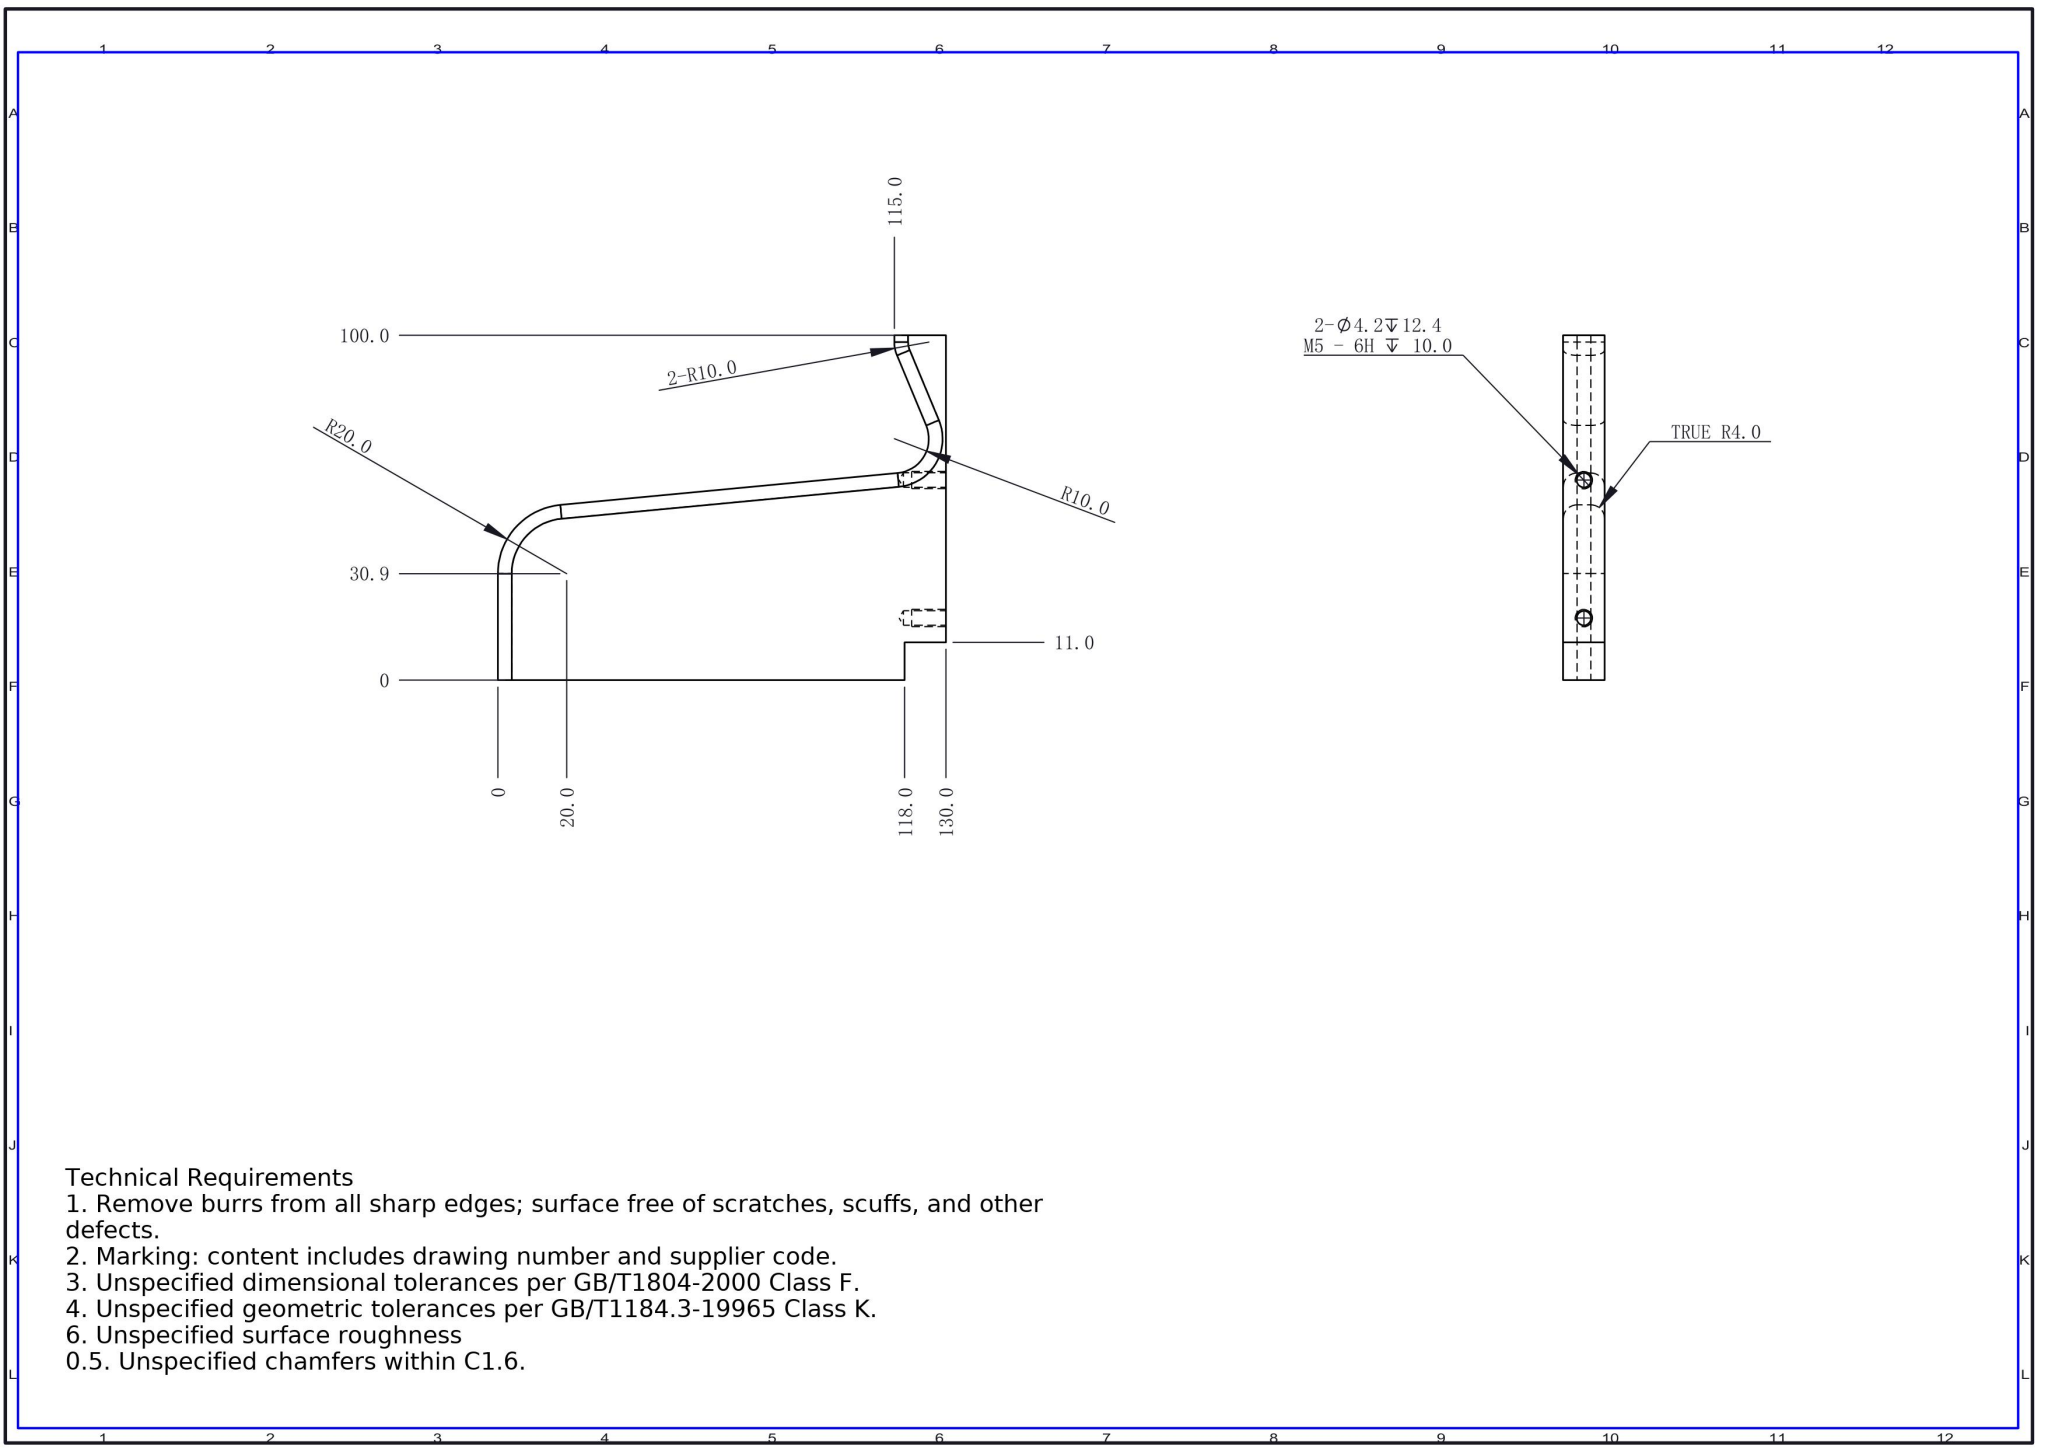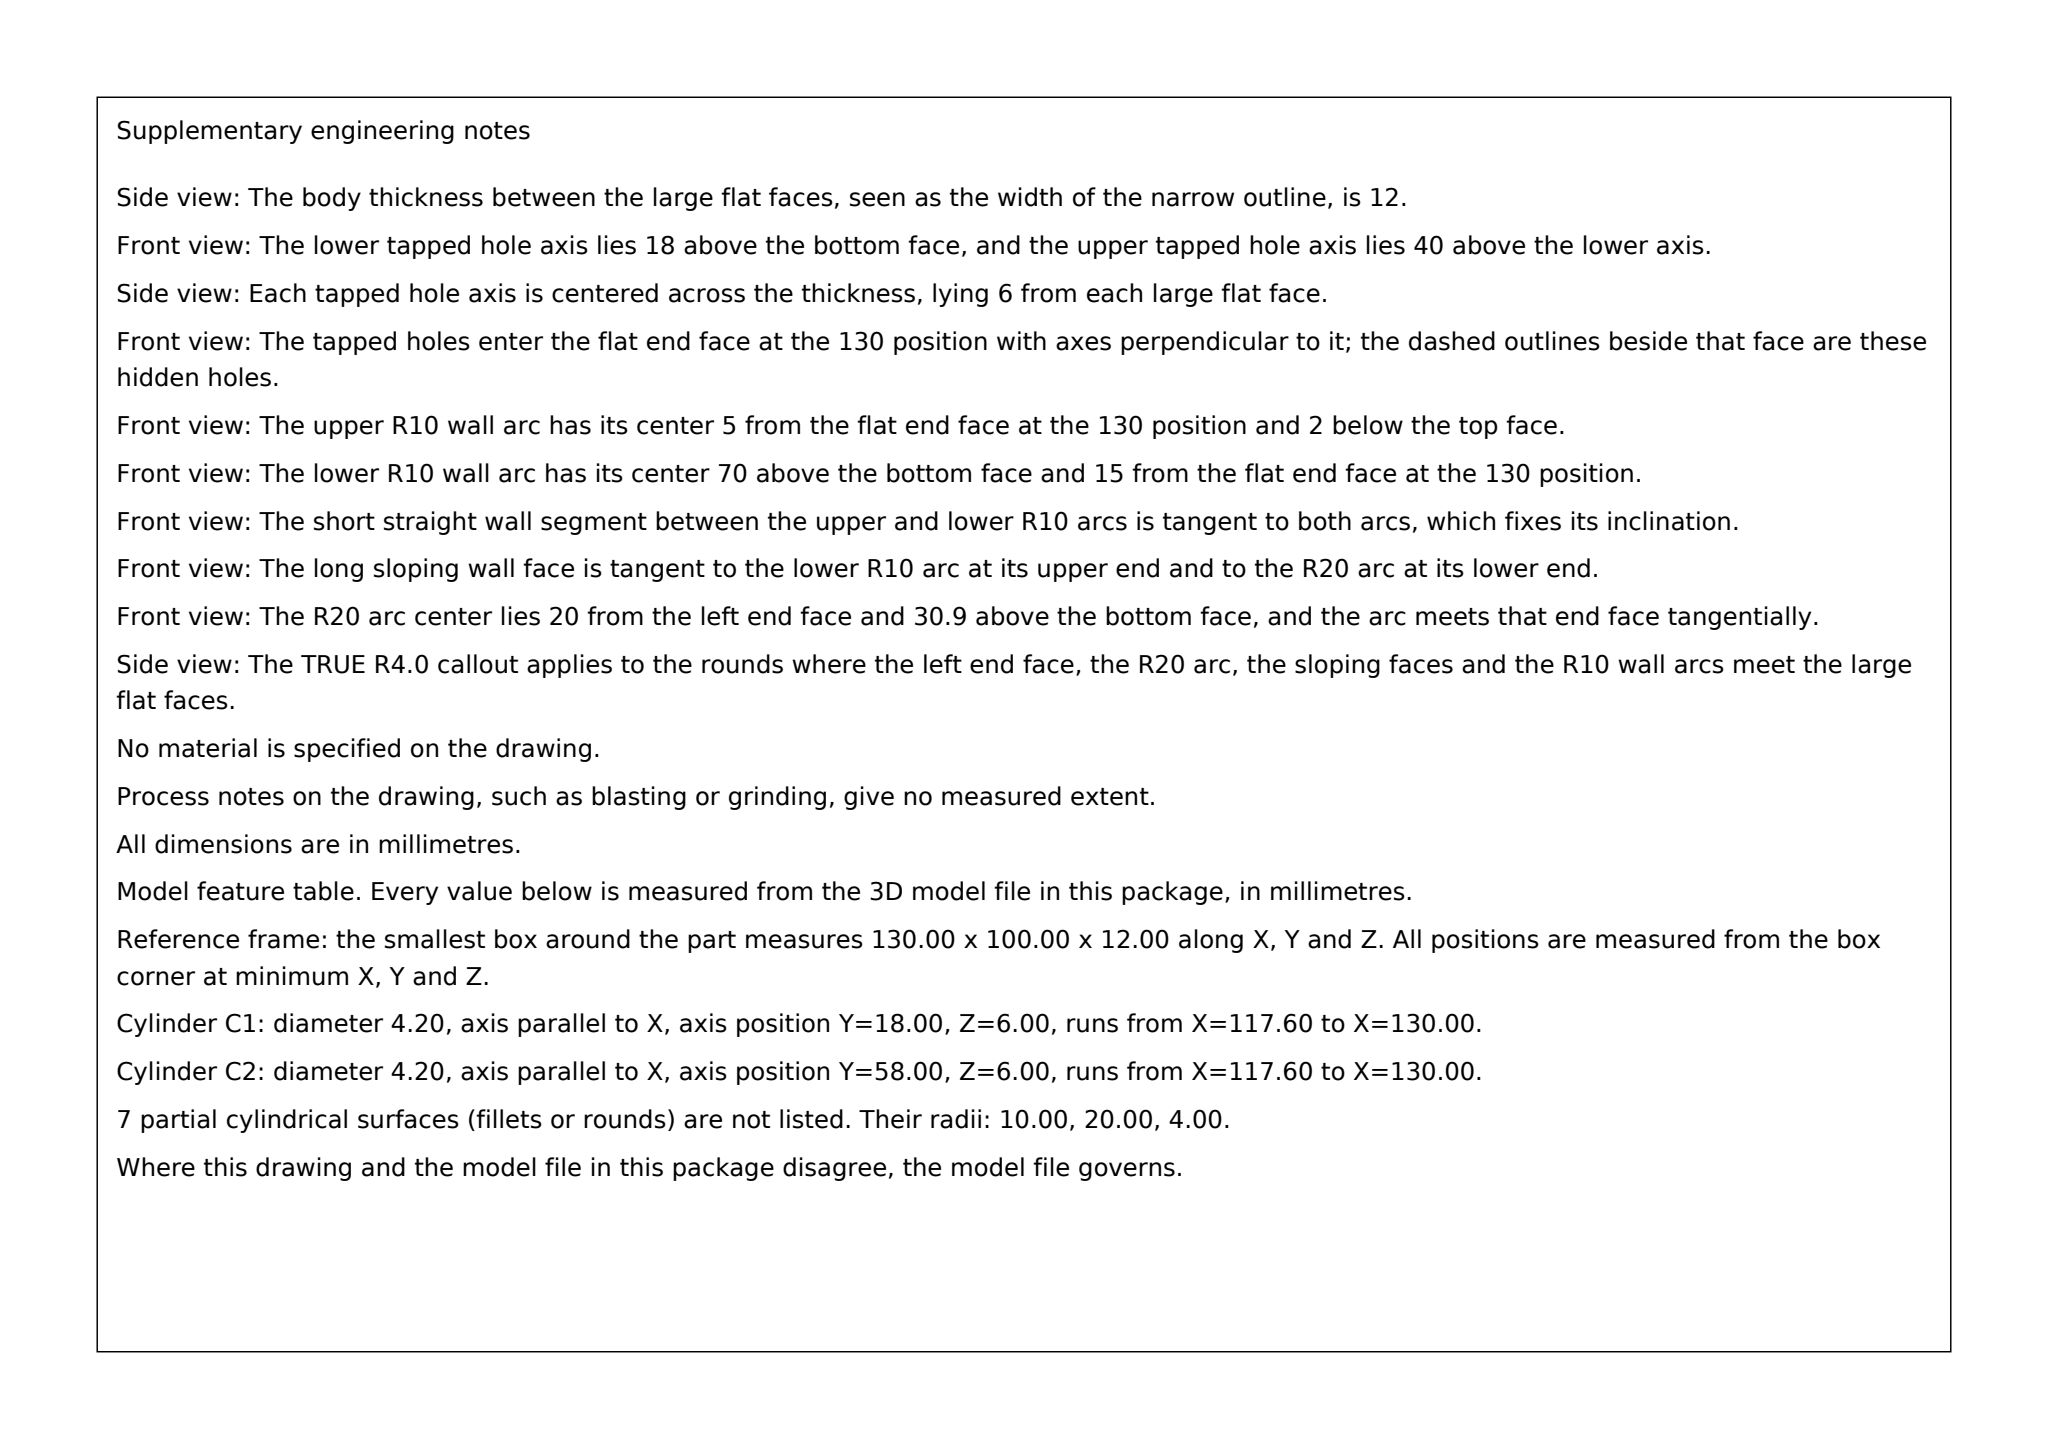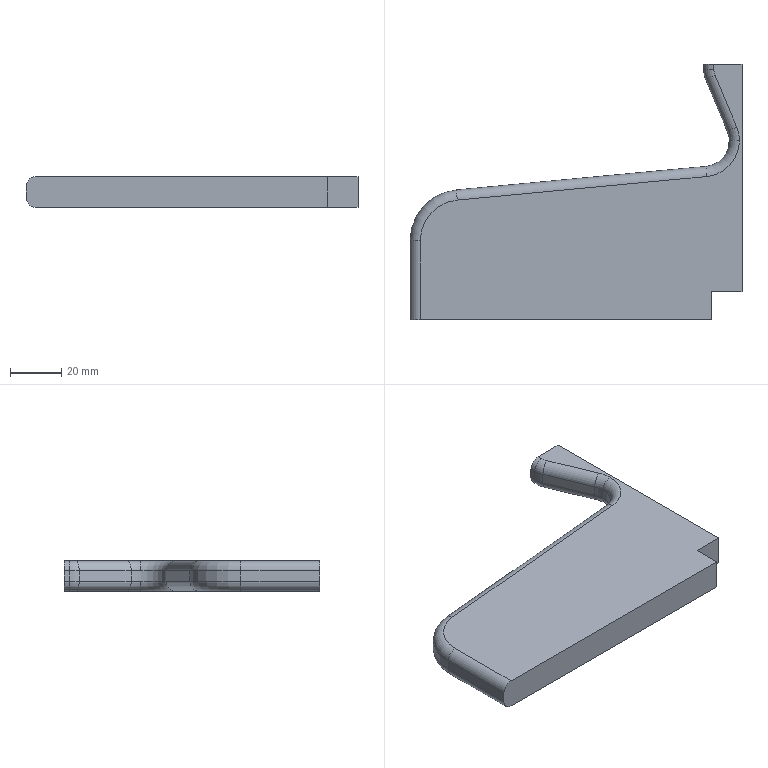Part | SolidWorks | mm | 1 solid | 38 faces | box 130 x 100 x 12 mm | volume 86452 mm3 | cylinder 15 | plane 11 | torus 8 | cone 4 | commonest cylinder face diameters 8 x8 4.2 x4 20 x2 40 x1
Drawing notes:
BAR SECTION 8.0 WIDE X 12.0 THK, TRUE R4.0 ENDS (TYP) | from the solid: Sweep profile from dia 8.0 corner cyls at z=4.0 & z=8.0, bbox z=12.0, fillet_radii 4.0 x8
UPPER R10.0 BEND CTR X=125.0; PART ENDS 3.225 PAST 130.0 | from the solid: 20.0 dia z-cyl ctr x=126.65,y=98.0 minus datum plane x=1.65 => 125.0; bbox x 134.875 - back face plane x=131.65 = 3.225